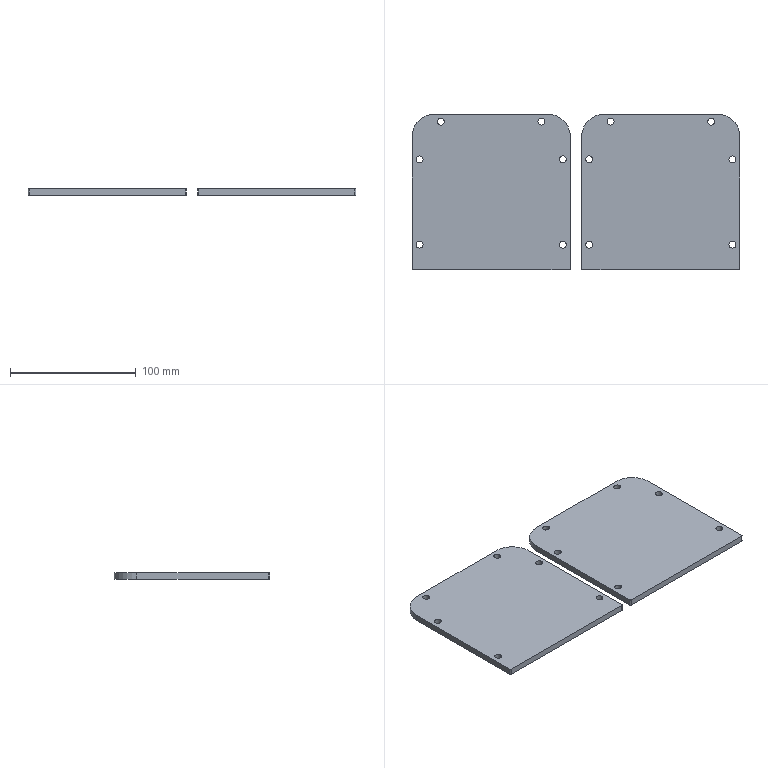CAM job | Mastercam | mm | 4 operations | part box 261 x 124 x 5
1. Contour (Ramp) | 3 - 3 平铣刀
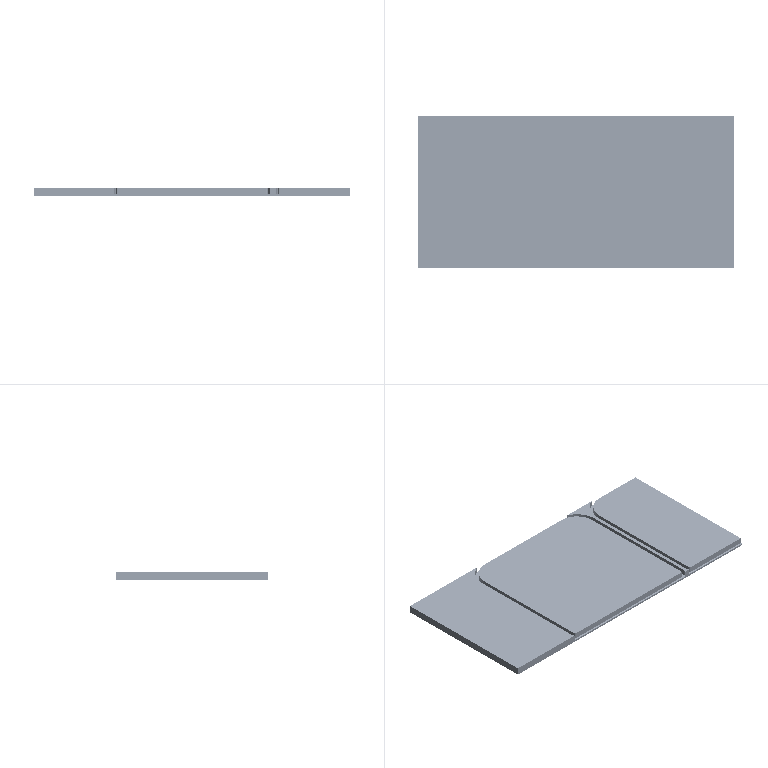2. Drill/Counterbore | 5 - 4 倒角刀
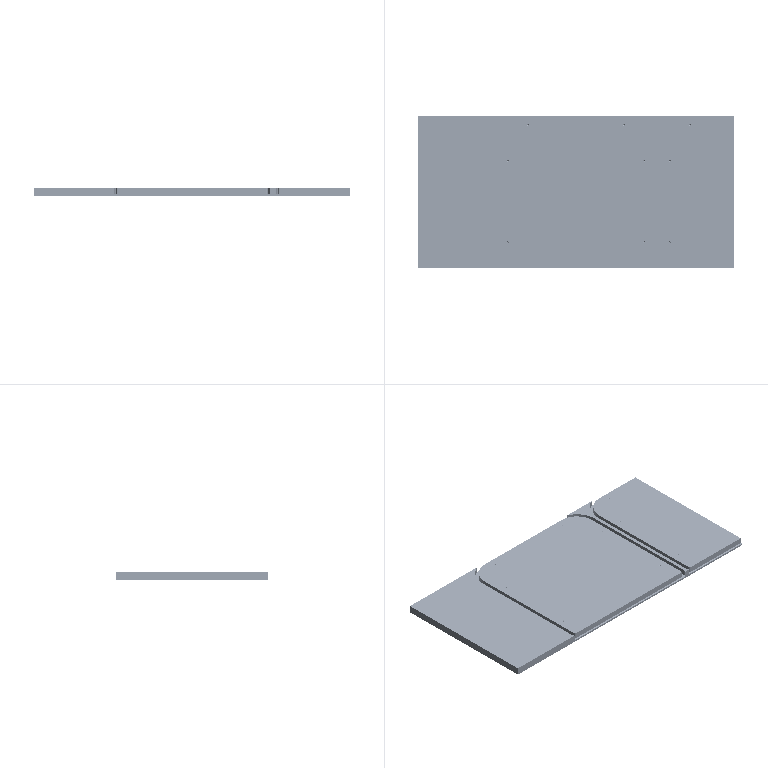3. Contour (2D chamfer) | 5 - 4 倒角刀
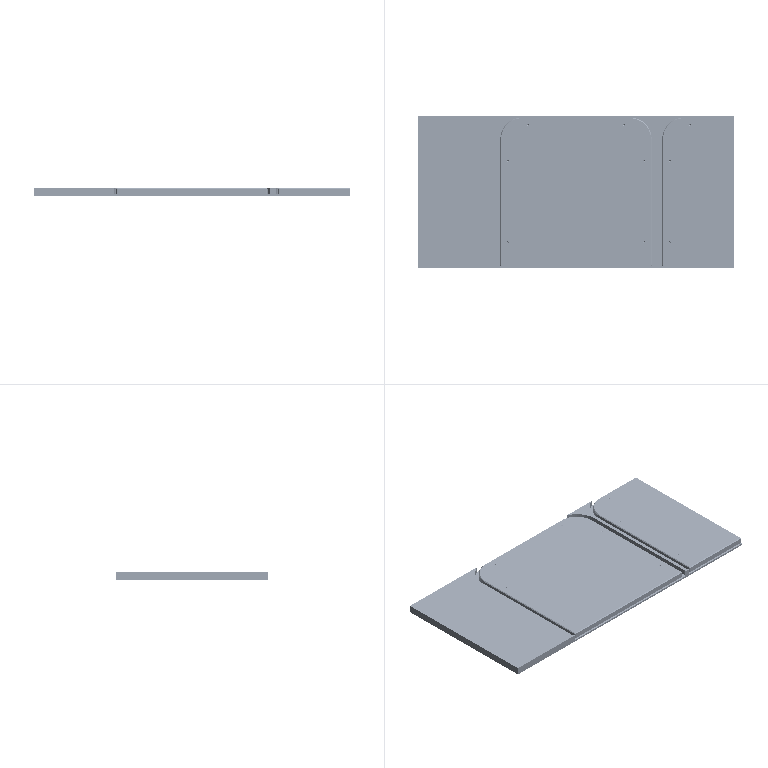4. Contour (Ramp) | 2 - 2 平铣刀